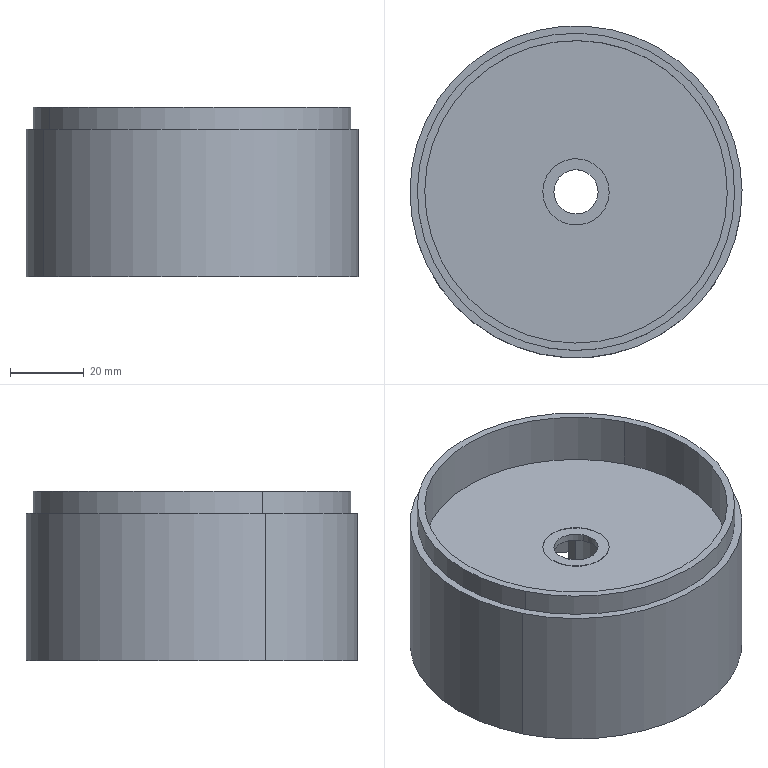Component | SolidWorks | g2-1 | 1 solid | 33 faces | box 90 x 90 x 46 mm | volume 53893 mm3 | cylinder 20 | plane 13 | commonest cylinder face diameters 18 x5 86 x4 82 x4 22 x3 12 x2 90 x2
build123d program:
from build123d import *
from build123d.topology import SkipClean

# Parameters (mm, degrees)
SKETCH1_2_R             = 45
SKETCH1_2_R_2           = 41
BOSS_EXTRUDE1_DEPTH     = 20
BOSS_EXTRUDE2_2_START   = 6
SKETCH2_2_R             = 43
SKETCH2_2_R_2           = 41
BOSS_EXTRUDE2_2_DEPTH   = 6
SKETCH3_W               = 3
SKETCH3_H               = 4.784
SKETCH4_2_W             = 2
SKETCH4_2_H             = 36
BOSS_EXTRUDE3_START     = 16
SKETCH5_R               = 11
SKETCH5_R_2             = 9
BOSS_EXTRUDE3_DEPTH     = 16
BOSS_EXTRUDE4_START     = 2
SKETCH6_R               = 11
SKETCH6_R_2             = 6
BOSS_EXTRUDE4_DEPTH     = 2
CUT_EXTRUDE1_START      = -8
SKETCH1_R               = 43
CUT_EXTRUDE1_DEPTH      = 8
CUT_EXTRUDE2_DEPTH      = 10
CUT_EXTRUDE2_DEPTH_BACK = 10
BOSS_EXTRUDE2_START     = -10
SKETCH4_R               = 9
SKETCH4_R_2             = 6
BOSS_EXTRUDE2_DEPTH     = 1.9


with BuildPart() as part:
    # Sketch1_2 → Boss-Extrude1 (new, symmetric)
    with BuildSketch(Plane.XY):
        Circle(SKETCH1_2_R)
        Circle(SKETCH1_2_R_2, mode=Mode.SUBTRACT)
    extrude(amount=BOSS_EXTRUDE1_DEPTH, both=True)

    # Sketch2_2 → Boss-Extrude2_2 (add)
    with SkipClean():  # the faces are left unmerged after this step: merging them gives an invalid solid
        with BuildSketch(Plane(origin=(0, 0, -20), x_dir=(-1, 0, 0), z_dir=(0, 0, -1)).offset(BOSS_EXTRUDE2_2_START)):
            with Locations(Location((0, 0, 0), (0, 0, 180))):
                Circle(SKETCH2_2_R)
            Circle(SKETCH2_2_R_2, mode=Mode.SUBTRACT)
        extrude(amount=-BOSS_EXTRUDE2_2_DEPTH)

    # Sketch3 → Cut-Revolve2 (revolve, cut)
    with BuildSketch(Plane(origin=(0, 0, 0), x_dir=(0, 0, -1), z_dir=(1, 0, 0)), mode=Mode.PRIVATE) as cut_revolve2_sk:
        with Locations((-18.5, 40.608)):
            Rectangle(SKETCH3_W, SKETCH3_H)
    revolve(cut_revolve2_sk.sketch.rotate(Axis((0, 0, 50.051), (0, 0, -1)), 270), axis=Axis((0, 0, 50.051), (0, 0, -1)), mode=Mode.SUBTRACT)

    # Sketch4_2 → Revolve1 (revolve)
    with BuildSketch(Plane(origin=(0, 0, 0), x_dir=(0, 0, -1), z_dir=(1, 0, 0)), mode=Mode.PRIVATE) as revolve1_sk:
        with Locations((11, 27)):
            Rectangle(SKETCH4_2_W, SKETCH4_2_H)
    revolve(revolve1_sk.sketch.rotate(Axis((0, 0, 44.645), (0, 0, -1)), 270), axis=Axis((0, 0, 44.645), (0, 0, -1)))

    # Sketch5 → Boss-Extrude3 (add)
    with BuildSketch(Plane.XY.offset(-10).offset(BOSS_EXTRUDE3_START)):
        with Locations(Location((0, 0, 0), (0, 0, 180))):
            Circle(SKETCH5_R)
        Circle(SKETCH5_R_2, mode=Mode.SUBTRACT)
    extrude(amount=-BOSS_EXTRUDE3_DEPTH)

    # Sketch6 → Boss-Extrude4 (add)
    with BuildSketch(Plane.XY.offset(6).offset(BOSS_EXTRUDE4_START)):
        with Locations(Location((0, 0, 0), (0, 0, 180))):
            Circle(SKETCH6_R)
        Circle(SKETCH6_R_2, mode=Mode.SUBTRACT)
    extrude(amount=-BOSS_EXTRUDE4_DEPTH)

    # Sketch1 → Cut-Extrude1 (cut)
    with BuildSketch(Plane.XY.offset(20).offset(CUT_EXTRUDE1_START)):
        Circle(SKETCH1_R)
    extrude(amount=CUT_EXTRUDE1_DEPTH, mode=Mode.SUBTRACT)

    # Sketch2 → Cut-Extrude2 (cut, two sides: drawn at the far end of the back side and taken through both)
    with BuildSketch(Plane.XY.offset(-CUT_EXTRUDE2_DEPTH_BACK)):
        Polygon((-18.876, 24.127), (7.766, -29.633), (18.876, -24.127), (-7.766, 29.633), align=None)
    extrude(amount=CUT_EXTRUDE2_DEPTH + CUT_EXTRUDE2_DEPTH_BACK, mode=Mode.SUBTRACT)

    # Sketch4 → Boss-Extrude2 (add)
    with BuildSketch(Plane.XY.offset(BOSS_EXTRUDE2_START)):
        Circle(SKETCH4_R)
        Circle(SKETCH4_R_2, mode=Mode.SUBTRACT)
    extrude(amount=-BOSS_EXTRUDE2_DEPTH)


solid = part.part

# Placed as in the assembly
solid = solid.moved(Location((-15.928, -1.7, 148), (-180, 0, -26.361)))
STEP:
#1=CARTESIAN_POINT('',(-0.4154,0.03795,6.295));
#2=VERTEX_POINT('',#1);
#3=CARTESIAN_POINT('',(-0.8387,-0.1718,6.295));
#4=VERTEX_POINT('',#3);
#5=CARTESIAN_POINT('',(-0.6271,-0.06694,6.295));
#6=DIRECTION('',(0.,0.,-1.));
#7=DIRECTION('',(-0.896,-0.444,0.));
#8=AXIS2_PLACEMENT_3D('',#5,#6,#7);
#9=CIRCLE('',#8,0.2362);
#10=EDGE_CURVE('',#2,#4,#9,.T.);
#11=ORIENTED_EDGE('',*,*,#10,.F.);
#12=CARTESIAN_POINT('',(-0.4154,0.03795,6.22));
#13=VERTEX_POINT('',#12);
#14=CARTESIAN_POINT('',(-0.4154,0.03795,6.295));
#15=DIRECTION('',(0.,0.,-1.));
#16=VECTOR('',#15,39.37);
#17=LINE('',#14,#16);
#18=EDGE_CURVE('',#2,#13,#17,.T.);
#19=ORIENTED_EDGE('',*,*,#18,.T.);
#20=CARTESIAN_POINT('',(-0.8387,-0.1718,6.22));
#21=VERTEX_POINT('',#20);
#22=CARTESIAN_POINT('',(-0.6271,-0.06694,6.22));
#23=DIRECTION('',(0.,0.,-1.));
#24=DIRECTION('',(-0.896,-0.444,0.));
#25=AXIS2_PLACEMENT_3D('',#22,#23,#24);
#26=CIRCLE('',#25,0.2362);
#27=EDGE_CURVE('',#13,#21,#26,.T.);
#28=ORIENTED_EDGE('',*,*,#27,.T.);
#29=CARTESIAN_POINT('',(-0.8387,-0.1718,6.295));
#30=DIRECTION('',(0.,0.,-1.));
#31=VECTOR('',#30,39.37);
#32=LINE('',#29,#31);
#33=EDGE_CURVE('',#4,#21,#32,.T.);
#34=ORIENTED_EDGE('',*,*,#33,.F.);
#35=EDGE_LOOP('',(#11,#19,#28,#34));
#36=FACE_OUTER_BOUND('',#35,.T.);
#37=CARTESIAN_POINT('',(-0.6271,-0.06694,6.295));
#38=DIRECTION('',(0.,0.,-1.));
#39=DIRECTION('',(-0.896,-0.444,0.));
#40=AXIS2_PLACEMENT_3D('',#37,#38,#39);
#41=CYLINDRICAL_SURFACE('',#40,0.2362);
#42=ADVANCED_FACE('',(#36),#41,.F.);
#43=CARTESIAN_POINT('',(0.8898,0.6848,5.354));
#44=VERTEX_POINT('',#43);
#45=CARTESIAN_POINT('',(-2.144,-0.8186,5.354));
#46=VERTEX_POINT('',#45);
#47=CARTESIAN_POINT('',(-0.6271,-0.06694,5.354));
#48=DIRECTION('',(0.,0.,-1.));
#49=DIRECTION('',(-0.896,-0.444,0.));
#50=AXIS2_PLACEMENT_3D('',#47,#48,#49);
#51=CIRCLE('',#50,1.693);
#52=EDGE_CURVE('',#44,#46,#51,.T.);
#53=ORIENTED_EDGE('',*,*,#52,.F.);
#54=CARTESIAN_POINT('',(0.8898,0.6848,5.039));
#55=VERTEX_POINT('',#54);
#56=CARTESIAN_POINT('',(0.8898,0.6848,3.856));
#57=DIRECTION('',(0.,0.,-1.));
#58=VECTOR('',#57,39.37);
#59=LINE('',#56,#58);
#60=EDGE_CURVE('',#44,#55,#59,.T.);
#61=ORIENTED_EDGE('',*,*,#60,.T.);
#62=CARTESIAN_POINT('',(-2.144,-0.8186,5.039));
#63=VERTEX_POINT('',#62);
#64=CARTESIAN_POINT('',(-0.6271,-0.06694,5.039));
#65=DIRECTION('',(0.,0.,-1.));
#66=DIRECTION('',(-0.896,-0.444,0.));
#67=AXIS2_PLACEMENT_3D('',#64,#65,#66);
#68=CIRCLE('',#67,1.693);
#69=EDGE_CURVE('',#55,#63,#68,.T.);
#70=ORIENTED_EDGE('',*,*,#69,.T.);
#71=CARTESIAN_POINT('',(-2.144,-0.8186,3.856));
#72=DIRECTION('',(0.,0.,-1.));
#73=VECTOR('',#72,39.37);
#74=LINE('',#71,#73);
#75=EDGE_CURVE('',#46,#63,#74,.T.);
#76=ORIENTED_EDGE('',*,*,#75,.F.);
#77=EDGE_LOOP('',(#53,#61,#70,#76));
#78=FACE_OUTER_BOUND('',#77,.T.);
#79=CARTESIAN_POINT('',(-0.6271,-0.06694,3.856));
#80=DIRECTION('',(0.,0.,-1.));
#81=DIRECTION('',(-0.896,-0.444,0.));
#82=AXIS2_PLACEMENT_3D('',#79,#80,#81);
#83=CYLINDRICAL_SURFACE('',#82,1.693);
#84=ADVANCED_FACE('',(#78),#83,.F.);
#85=CARTESIAN_POINT('',(0.8898,0.6848,6.85));
#86=VERTEX_POINT('',#85);
#87=CARTESIAN_POINT('',(-2.144,-0.8186,6.85));
#88=VERTEX_POINT('',#87);
#89=CARTESIAN_POINT('',(-0.6271,-0.06694,6.85));
#90=DIRECTION('',(0.,0.,1.));
#91=DIRECTION('',(0.896,0.444,0.));
#92=AXIS2_PLACEMENT_3D('',#89,#90,#91);
#93=CIRCLE('',#92,1.693);
#94=EDGE_CURVE('',#86,#88,#93,.T.);
#95=ORIENTED_EDGE('',*,*,#94,.F.);
#96=CARTESIAN_POINT('',(0.8898,0.6848,6.614));
#97=VERTEX_POINT('',#96);
#98=CARTESIAN_POINT('',(0.8898,0.6848,6.85));
#99=DIRECTION('',(0.,0.,-1.));
#100=VECTOR('',#99,39.37);
#101=LINE('',#98,#100);
#102=EDGE_CURVE('',#86,#97,#101,.T.);
#103=ORIENTED_EDGE('',*,*,#102,.T.);
#104=CARTESIAN_POINT('',(-2.144,-0.8186,6.614));
#105=VERTEX_POINT('',#104);
#106=CARTESIAN_POINT('',(-0.6271,-0.06694,6.614));
#107=DIRECTION('',(0.,0.,1.));
#108=DIRECTION('',(-0.896,-0.444,0.));
#109=AXIS2_PLACEMENT_3D('',#106,#107,#108);
#110=CIRCLE('',#109,1.693);
#111=EDGE_CURVE('',#97,#105,#110,.T.);
#112=ORIENTED_EDGE('',*,*,#111,.T.);
#113=CARTESIAN_POINT('',(-2.144,-0.8186,6.85));
#114=DIRECTION('',(0.,0.,-1.));
#115=VECTOR('',#114,39.37);
#116=LINE('',#113,#115);
#117=EDGE_CURVE('',#88,#105,#116,.T.);
#118=ORIENTED_EDGE('',*,*,#117,.F.);
#119=EDGE_LOOP('',(#95,#103,#112,#118));
#120=FACE_OUTER_BOUND('',#119,.T.);
#121=CARTESIAN_POINT('',(-0.6271,-0.06694,6.85));
#122=DIRECTION('',(0.,0.,-1.));
#123=DIRECTION('',(-0.896,-0.444,0.));
#124=AXIS2_PLACEMENT_3D('',#121,#122,#123);
#125=CYLINDRICAL_SURFACE('',#124,1.693);
#126=ADVANCED_FACE('',(#120),#125,.T.);
#127=CARTESIAN_POINT('',(-2.215,-0.8536,5.039));
#128=VERTEX_POINT('',#127);
#129=CARTESIAN_POINT('',(0.9603,0.7197,5.039));
#130=VERTEX_POINT('',#129);
#131=CARTESIAN_POINT('',(-0.6271,-0.06694,5.039));
#132=DIRECTION('',(0.,0.,-1.));
#133=DIRECTION('',(-0.896,-0.444,0.));
#134=AXIS2_PLACEMENT_3D('',#131,#132,#133);
#135=CIRCLE('',#134,1.772);
#136=EDGE_CURVE('',#128,#130,#135,.T.);
#137=ORIENTED_EDGE('',*,*,#136,.F.);
#138=CARTESIAN_POINT('',(-2.215,-0.8536,6.614));
#139=VERTEX_POINT('',#138);
#140=CARTESIAN_POINT('',(-2.215,-0.8536,5.039));
#141=DIRECTION('',(0.,0.,1.));
#142=VECTOR('',#141,39.37);
#143=LINE('',#140,#142);
#144=EDGE_CURVE('',#128,#139,#143,.T.);
#145=ORIENTED_EDGE('',*,*,#144,.T.);
#146=CARTESIAN_POINT('',(0.9603,0.7197,6.614));
#147=VERTEX_POINT('',#146);
#148=CARTESIAN_POINT('',(-0.6271,-0.06694,6.614));
#149=DIRECTION('',(0.,0.,-1.));
#150=DIRECTION('',(-0.896,-0.444,0.));
#151=AXIS2_PLACEMENT_3D('',#148,#149,#150);
#152=CIRCLE('',#151,1.772);
#153=EDGE_CURVE('',#139,#147,#152,.T.);
#154=ORIENTED_EDGE('',*,*,#153,.T.);
#155=CARTESIAN_POINT('',(0.9603,0.7197,5.039));
#156=DIRECTION('',(0.,0.,1.));
#157=VECTOR('',#156,39.37);
#158=LINE('',#155,#157);
#159=EDGE_CURVE('',#130,#147,#158,.T.);
#160=ORIENTED_EDGE('',*,*,#159,.F.);
#161=EDGE_LOOP('',(#137,#145,#154,#160));
#162=FACE_OUTER_BOUND('',#161,.T.);
#163=CARTESIAN_POINT('',(-0.6271,-0.06694,5.039));
#164=DIRECTION('',(0.,0.,1.));
#165=DIRECTION('',(0.896,0.444,0.));
#166=AXIS2_PLACEMENT_3D('',#163,#164,#165);
#167=CYLINDRICAL_SURFACE('',#166,1.772);
#168=ADVANCED_FACE('',(#162),#167,.T.);
#169=CARTESIAN_POINT('',(0.8192,0.6498,6.299));
#170=VERTEX_POINT('',#169);
#171=CARTESIAN_POINT('',(-2.073,-0.7837,6.299));
#172=VERTEX_POINT('',#171);
#173=CARTESIAN_POINT('',(-0.6271,-0.06694,6.299));
#174=DIRECTION('',(0.,0.,-1.));
#175=DIRECTION('',(-0.896,-0.444,0.));
#176=AXIS2_PLACEMENT_3D('',#173,#174,#175);
#177=CIRCLE('',#176,1.614);
#178=EDGE_CURVE('',#170,#172,#177,.T.);
#179=ORIENTED_EDGE('',*,*,#178,.T.);
#180=CARTESIAN_POINT('',(-2.073,-0.7837,6.85));
#181=VERTEX_POINT('',#180);
#182=CARTESIAN_POINT('',(-2.073,-0.7837,5.039));
#183=DIRECTION('',(0.,0.,1.));
#184=VECTOR('',#183,39.37);
#185=LINE('',#182,#184);
#186=EDGE_CURVE('',#172,#181,#185,.T.);
#187=ORIENTED_EDGE('',*,*,#186,.T.);
#188=CARTESIAN_POINT('',(0.8192,0.6498,6.85));
#189=VERTEX_POINT('',#188);
#190=CARTESIAN_POINT('',(-0.6271,-0.06694,6.85));
#191=DIRECTION('',(0.,0.,1.));
#192=DIRECTION('',(0.896,0.444,0.));
#193=AXIS2_PLACEMENT_3D('',#190,#191,#192);
#194=CIRCLE('',#193,1.614);
#195=EDGE_CURVE('',#181,#189,#194,.T.);
#196=ORIENTED_EDGE('',*,*,#195,.T.);
#197=CARTESIAN_POINT('',(0.8192,0.6498,5.039));
#198=DIRECTION('',(0.,0.,1.));
#199=VECTOR('',#198,39.37);
#200=LINE('',#197,#199);
#201=EDGE_CURVE('',#170,#189,#200,.T.);
#202=ORIENTED_EDGE('',*,*,#201,.F.);
#203=EDGE_LOOP('',(#179,#187,#196,#202));
#204=FACE_OUTER_BOUND('',#203,.T.);
#205=CARTESIAN_POINT('',(-0.6271,-0.06694,5.039));
#206=DIRECTION('',(0.,0.,1.));
#207=DIRECTION('',(0.896,0.444,0.));
#208=AXIS2_PLACEMENT_3D('',#205,#206,#207);
#209=CYLINDRICAL_SURFACE('',#208,1.614);
#210=ADVANCED_FACE('',(#204),#209,.F.);
#211=CARTESIAN_POINT('',(0.8192,0.6498,5.354));
#212=VERTEX_POINT('',#211);
#213=CARTESIAN_POINT('',(-2.073,-0.7837,5.354));
#214=VERTEX_POINT('',#213);
#215=CARTESIAN_POINT('',(-0.6271,-0.06694,5.354));
#216=DIRECTION('',(0.,0.,-1.));
#217=DIRECTION('',(-0.896,-0.444,0.));
#218=AXIS2_PLACEMENT_3D('',#215,#216,#217);
#219=CIRCLE('',#218,1.614);
#220=EDGE_CURVE('',#212,#214,#219,.T.);
#221=ORIENTED_EDGE('',*,*,#220,.T.);
#222=CARTESIAN_POINT('',(-2.073,-0.7837,6.22));
#223=VERTEX_POINT('',#222);
#224=CARTESIAN_POINT('',(-2.073,-0.7837,5.039));
#225=DIRECTION('',(0.,0.,1.));
#226=VECTOR('',#225,39.37);
#227=LINE('',#224,#226);
#228=EDGE_CURVE('',#214,#223,#227,.T.);
#229=ORIENTED_EDGE('',*,*,#228,.T.);
#230=CARTESIAN_POINT('',(0.8192,0.6498,6.22));
#231=VERTEX_POINT('',#230);
#232=CARTESIAN_POINT('',(-0.6271,-0.06694,6.22));
#233=DIRECTION('',(0.,0.,1.));
#234=DIRECTION('',(0.896,0.444,0.));
#235=AXIS2_PLACEMENT_3D('',#232,#233,#234);
#236=CIRCLE('',#235,1.614);
#237=EDGE_CURVE('',#223,#231,#236,.T.);
#238=ORIENTED_EDGE('',*,*,#237,.T.);
#239=CARTESIAN_POINT('',(0.8192,0.6498,5.039));
#240=DIRECTION('',(0.,0.,1.));
#241=VECTOR('',#240,39.37);
#242=LINE('',#239,#241);
#243=EDGE_CURVE('',#212,#231,#242,.T.);
#244=ORIENTED_EDGE('',*,*,#243,.F.);
#245=EDGE_LOOP('',(#221,#229,#238,#244));
#246=FACE_OUTER_BOUND('',#245,.T.);
#247=CARTESIAN_POINT('',(-0.6271,-0.06694,5.039));
#248=DIRECTION('',(0.,0.,1.));
#249=DIRECTION('',(0.896,0.444,0.));
#250=AXIS2_PLACEMENT_3D('',#247,#248,#249);
#251=CYLINDRICAL_SURFACE('',#250,1.614);
#252=ADVANCED_FACE('',(#246),#251,.F.);
#253=CARTESIAN_POINT('',(-0.2391,0.1254,5.512));
#254=VERTEX_POINT('',#253);
#255=CARTESIAN_POINT('',(-0.383,-0.4247,5.512));
#256=VERTEX_POINT('',#255);
#257=CARTESIAN_POINT('',(-0.6271,-0.06694,5.512));
#258=DIRECTION('',(0.,0.,-1.));
#259=DIRECTION('',(-0.896,-0.444,0.));
#260=AXIS2_PLACEMENT_3D('',#257,#258,#259);
#261=CIRCLE('',#260,0.4331);
#262=EDGE_CURVE('',#254,#256,#261,.T.);
#263=ORIENTED_EDGE('',*,*,#262,.F.);
#264=CARTESIAN_POINT('',(-0.2391,0.1254,6.22));
#265=VERTEX_POINT('',#264);
#266=CARTESIAN_POINT('',(-0.2391,0.1254,5.591));
#267=DIRECTION('',(0.,0.,1.));
#268=VECTOR('',#267,39.37);
#269=LINE('',#266,#268);
#270=EDGE_CURVE('',#254,#265,#269,.T.);
#271=ORIENTED_EDGE('',*,*,#270,.T.);
#272=CARTESIAN_POINT('',(-0.383,-0.4247,6.22));
#273=VERTEX_POINT('',#272);
#274=CARTESIAN_POINT('',(-0.6271,-0.06694,6.22));
#275=DIRECTION('',(0.,0.,-1.));
#276=DIRECTION('',(0.896,0.444,0.));
#277=AXIS2_PLACEMENT_3D('',#274,#275,#276);
#278=CIRCLE('',#277,0.4331);
#279=EDGE_CURVE('',#265,#273,#278,.T.);
#280=ORIENTED_EDGE('',*,*,#279,.T.);
#281=CARTESIAN_POINT('',(-0.383,-0.4247,5.591));
#282=DIRECTION('',(0.,0.,1.));
#283=VECTOR('',#282,39.37);
#284=LINE('',#281,#283);
#285=EDGE_CURVE('',#256,#273,#284,.T.);
#286=ORIENTED_EDGE('',*,*,#285,.F.);
#287=EDGE_LOOP('',(#263,#271,#280,#286));
#288=FACE_OUTER_BOUND('',#287,.T.);
#289=CARTESIAN_POINT('',(-0.6271,-0.06694,5.591));
#290=DIRECTION('',(0.,0.,1.));
#291=DIRECTION('',(0.896,0.444,0.));
#292=AXIS2_PLACEMENT_3D('',#289,#290,#291);
#293=CYLINDRICAL_SURFACE('',#292,0.4331);
#294=ADVANCED_FACE('',(#288),#293,.T.);
#295=CARTESIAN_POINT('',(-0.3096,0.0904,6.299));
#296=VERTEX_POINT('',#295);
#297=CARTESIAN_POINT('',(-0.9446,-0.2243,6.299));
#298=VERTEX_POINT('',#297);
#299=CARTESIAN_POINT('',(-0.6271,-0.06694,6.299));
#300=DIRECTION('',(0.,0.,-1.));
#301=DIRECTION('',(-0.896,-0.444,0.));
#302=AXIS2_PLACEMENT_3D('',#299,#300,#301);
#303=CIRCLE('',#302,0.3543);
#304=EDGE_CURVE('',#296,#298,#303,.T.);
#305=ORIENTED_EDGE('',*,*,#304,.F.);
#306=CARTESIAN_POINT('',(-0.3096,0.0904,6.295));
#307=VERTEX_POINT('',#306);
#308=CARTESIAN_POINT('',(-0.3096,0.0904,4.069));
#309=DIRECTION('',(0.,0.,-1.));
#310=VECTOR('',#309,39.37);
#311=LINE('',#308,#310);
#312=EDGE_CURVE('',#296,#307,#311,.T.);
#313=ORIENTED_EDGE('',*,*,#312,.T.);
#314=CARTESIAN_POINT('',(-0.9446,-0.2243,6.295));
#315=VERTEX_POINT('',#314);
#316=CARTESIAN_POINT('',(-0.6271,-0.06694,6.295));
#317=DIRECTION('',(0.,0.,1.));
#318=DIRECTION('',(-0.896,-0.444,0.));
#319=AXIS2_PLACEMENT_3D('',#316,#317,#318);
#320=CIRCLE('',#319,0.3543);
#321=EDGE_CURVE('',#315,#307,#320,.T.);
#322=ORIENTED_EDGE('',*,*,#321,.F.);
#323=CARTESIAN_POINT('',(-0.9446,-0.2243,4.069));
#324=DIRECTION('',(0.,0.,-1.));
#325=VECTOR('',#324,39.37);
#326=LINE('',#323,#325);
#327=EDGE_CURVE('',#298,#315,#326,.T.);
#328=ORIENTED_EDGE('',*,*,#327,.F.);
#329=EDGE_LOOP('',(#305,#313,#322,#328));
#330=FACE_OUTER_BOUND('',#329,.T.);
#331=CARTESIAN_POINT('',(-0.6271,-0.06694,4.069));
#332=DIRECTION('',(0.,0.,-1.));
#333=DIRECTION('',(-0.896,-0.444,0.));
#334=AXIS2_PLACEMENT_3D('',#331,#332,#333);
#335=CYLINDRICAL_SURFACE('',#334,0.3543);
#336=ADVANCED_FACE('',(#330),#335,.F.);
#337=CARTESIAN_POINT('',(-0.9446,-0.2243,6.22));
#338=VERTEX_POINT('',#337);
#339=CARTESIAN_POINT('',(-0.8712,0.1899,6.22));
#340=VERTEX_POINT('',#339);
#341=CARTESIAN_POINT('',(-0.6271,-0.06694,6.22));
#342=DIRECTION('',(0.,0.,-1.));
#343=DIRECTION('',(-0.896,-0.444,0.));
#344=AXIS2_PLACEMENT_3D('',#341,#342,#343);
#345=CIRCLE('',#344,0.3543);
#346=EDGE_CURVE('',#338,#340,#345,.T.);
#347=ORIENTED_EDGE('',*,*,#346,.F.);
#348=CARTESIAN_POINT('',(-0.9446,-0.2243,5.591));
#349=VERTEX_POINT('',#348);
#350=CARTESIAN_POINT('',(-0.9446,-0.2243,4.069));
#351=DIRECTION('',(0.,0.,-1.));
#352=VECTOR('',#351,39.37);
#353=LINE('',#350,#352);
#354=EDGE_CURVE('',#338,#349,#353,.T.);
#355=ORIENTED_EDGE('',*,*,#354,.T.);
#356=CARTESIAN_POINT('',(-0.8712,0.1899,5.591));
#357=VERTEX_POINT('',#356);
#358=CARTESIAN_POINT('',(-0.6271,-0.06694,5.591));
#359=DIRECTION('',(0.,0.,1.));
#360=DIRECTION('',(-0.896,-0.444,0.));
#361=AXIS2_PLACEMENT_3D('',#358,#359,#360);
#362=CIRCLE('',#361,0.3543);
#363=EDGE_CURVE('',#357,#349,#362,.T.);
#364=ORIENTED_EDGE('',*,*,#363,.F.);
#365=CARTESIAN_POINT('',(-0.8712,0.1899,4.069));
#366=DIRECTION('',(0.,0.,-1.));
#367=VECTOR('',#366,39.37);
#368=LINE('',#365,#367);
#369=EDGE_CURVE('',#340,#357,#368,.T.);
#370=ORIENTED_EDGE('',*,*,#369,.F.);
#371=EDGE_LOOP('',(#347,#355,#364,#370));
#372=FACE_OUTER_BOUND('',#371,.T.);
#373=CARTESIAN_POINT('',(-0.6271,-0.06694,4.069));
#374=DIRECTION('',(0.,0.,-1.));
#375=DIRECTION('',(-0.896,-0.444,0.));
#376=AXIS2_PLACEMENT_3D('',#373,#374,#375);
#377=CYLINDRICAL_SURFACE('',#376,0.3543);
#378=ADVANCED_FACE('',(#372),#377,.F.);
#379=CARTESIAN_POINT('',(-0.383,0.1899,6.22));
#380=VERTEX_POINT('',#379);
#381=CARTESIAN_POINT('',(-0.383,-0.3238,6.22));
#382=VERTEX_POINT('',#381);
#383=CARTESIAN_POINT('',(-0.6271,-0.06694,6.22));
#384=DIRECTION('',(0.,0.,-1.));
#385=DIRECTION('',(-0.896,-0.444,0.));
#386=AXIS2_PLACEMENT_3D('',#383,#384,#385);
#387=CIRCLE('',#386,0.3543);
#388=EDGE_CURVE('',#380,#382,#387,.T.);
#389=ORIENTED_EDGE('',*,*,#388,.F.);
#390=CARTESIAN_POINT('',(-0.383,0.1899,5.591));
#391=VERTEX_POINT('',#390);
#392=CARTESIAN_POINT('',(-0.383,0.1899,4.069));
#393=DIRECTION('',(0.,0.,1.));
#394=VECTOR('',#393,39.37);
#395=LINE('',#392,#394);
#396=EDGE_CURVE('',#391,#380,#395,.T.);
#397=ORIENTED_EDGE('',*,*,#396,.F.);
#398=CARTESIAN_POINT('',(-0.383,-0.3238,5.591));
#399=VERTEX_POINT('',#398);
#400=CARTESIAN_POINT('',(-0.6271,-0.06694,5.591));
#401=DIRECTION('',(0.,0.,1.));
#402=DIRECTION('',(-0.896,-0.444,0.));
#403=AXIS2_PLACEMENT_3D('',#400,#401,#402);
#404=CIRCLE('',#403,0.3543);
#405=EDGE_CURVE('',#399,#391,#404,.T.);
#406=ORIENTED_EDGE('',*,*,#405,.F.);
#407=CARTESIAN_POINT('',(-0.383,-0.3238,4.069));
#408=DIRECTION('',(0.,0.,-1.));
#409=VECTOR('',#408,39.37);
#410=LINE('',#407,#409);
#411=EDGE_CURVE('',#382,#399,#410,.T.);
#412=ORIENTED_EDGE('',*,*,#411,.F.);
#413=EDGE_LOOP('',(#389,#397,#406,#412));
#414=FACE_OUTER_BOUND('',#413,.T.);
#415=CARTESIAN_POINT('',(-0.6271,-0.06694,4.069));
#416=DIRECTION('',(0.,0.,-1.));
#417=DIRECTION('',(-0.896,-0.444,0.));
#418=AXIS2_PLACEMENT_3D('',#415,#416,#417);
#419=CYLINDRICAL_SURFACE('',#418,0.3543);
#420=ADVANCED_FACE('',(#414),#419,.F.);
#421=ORIENTED_EDGE('',*,*,#354,.F.);
#422=CARTESIAN_POINT('',(-0.8712,-0.3238,6.22));
#423=VERTEX_POINT('',#422);
#424=CARTESIAN_POINT('',(-0.6271,-0.06694,6.22));
#425=DIRECTION('',(0.,0.,-1.));
#426=DIRECTION('',(-0.896,-0.444,0.));
#427=AXIS2_PLACEMENT_3D('',#424,#425,#426);
#428=CIRCLE('',#427,0.3543);
#429=EDGE_CURVE('',#423,#338,#428,.T.);
#430=ORIENTED_EDGE('',*,*,#429,.F.);
#431=CARTESIAN_POINT('',(-0.8712,-0.3238,5.591));
#432=VERTEX_POINT('',#431);
#433=CARTESIAN_POINT('',(-0.8712,-0.3238,4.069));
#434=DIRECTION('',(0.,0.,1.));
#435=VECTOR('',#434,39.37);
#436=LINE('',#433,#435);
#437=EDGE_CURVE('',#432,#423,#436,.T.);
#438=ORIENTED_EDGE('',*,*,#437,.F.);
#439=CARTESIAN_POINT('',(-0.6271,-0.06694,5.591));
#440=DIRECTION('',(0.,0.,1.));
#441=DIRECTION('',(-0.896,-0.444,0.));
#442=AXIS2_PLACEMENT_3D('',#439,#440,#441);
#443=CIRCLE('',#442,0.3543);
#444=EDGE_CURVE('',#349,#432,#443,.T.);
#445=ORIENTED_EDGE('',*,*,#444,.F.);
#446=EDGE_LOOP('',(#421,#430,#438,#445));
#447=FACE_OUTER_BOUND('',#446,.T.);
#448=CARTESIAN_POINT('',(-0.6271,-0.06694,4.069));
#449=DIRECTION('',(0.,0.,-1.));
#450=DIRECTION('',(-0.896,-0.444,0.));
#451=AXIS2_PLACEMENT_3D('',#448,#449,#450);
#452=CYLINDRICAL_SURFACE('',#451,0.3543);
#453=ADVANCED_FACE('',(#447),#452,.F.);
#454=ORIENTED_EDGE('',*,*,#312,.F.);
#455=CARTESIAN_POINT('',(-0.6271,-0.06694,6.299));
#456=DIRECTION('',(0.,0.,-1.));
#457=DIRECTION('',(-0.896,-0.444,0.));
#458=AXIS2_PLACEMENT_3D('',#455,#456,#457);
#459=CIRCLE('',#458,0.3543);
#460=EDGE_CURVE('',#298,#296,#459,.T.);
#461=ORIENTED_EDGE('',*,*,#460,.F.);
#462=ORIENTED_EDGE('',*,*,#327,.T.);
#463=CARTESIAN_POINT('',(-0.6271,-0.06694,6.295));
#464=DIRECTION('',(0.,0.,1.));
#465=DIRECTION('',(-0.896,-0.444,0.));
#466=AXIS2_PLACEMENT_3D('',#463,#464,#465);
#467=CIRCLE('',#466,0.3543);
#468=EDGE_CURVE('',#307,#315,#467,.T.);
#469=ORIENTED_EDGE('',*,*,#468,.F.);
#470=EDGE_LOOP('',(#454,#461,#462,#469));
#471=FACE_OUTER_BOUND('',#470,.T.);
#472=CARTESIAN_POINT('',(-0.6271,-0.06694,4.069));
#473=DIRECTION('',(0.,0.,-1.));
#474=DIRECTION('',(-0.896,-0.444,0.));
#475=AXIS2_PLACEMENT_3D('',#472,#473,#474);
#476=CYLINDRICAL_SURFACE('',#475,0.3543);
#477=ADVANCED_FACE('',(#471),#476,.F.);
#478=ORIENTED_EDGE('',*,*,#270,.F.);
#479=CARTESIAN_POINT('',(-0.383,0.2908,5.512));
#480=VERTEX_POINT('',#479);
#481=CARTESIAN_POINT('',(-0.6271,-0.06694,5.512));
#482=DIRECTION('',(0.,0.,-1.));
#483=DIRECTION('',(-0.896,-0.444,0.));
#484=AXIS2_PLACEMENT_3D('',#481,#482,#483);
#485=CIRCLE('',#484,0.4331);
#486=EDGE_CURVE('',#480,#254,#485,.T.);
#487=ORIENTED_EDGE('',*,*,#486,.F.);
#488=CARTESIAN_POINT('',(-0.383,0.2908,6.22));
#489=VERTEX_POINT('',#488);
#490=CARTESIAN_POINT('',(-0.383,0.2908,5.591));
#491=DIRECTION('',(0.,0.,-1.));
#492=VECTOR('',#491,39.37);
#493=LINE('',#490,#492);
#494=EDGE_CURVE('',#489,#480,#493,.T.);
#495=ORIENTED_EDGE('',*,*,#494,.F.);
#496=CARTESIAN_POINT('',(-0.6271,-0.06694,6.22));
#497=DIRECTION('',(0.,0.,-1.));
#498=DIRECTION('',(0.896,0.444,0.));
#499=AXIS2_PLACEMENT_3D('',#496,#497,#498);
#500=CIRCLE('',#499,0.4331);
#501=EDGE_CURVE('',#489,#265,#500,.T.);
#502=ORIENTED_EDGE('',*,*,#501,.T.);
#503=EDGE_LOOP('',(#478,#487,#495,#502));
#504=FACE_OUTER_BOUND('',#503,.T.);
#505=CARTESIAN_POINT('',(-0.6271,-0.06694,5.591));
#506=DIRECTION('',(0.,0.,1.));
#507=DIRECTION('',(0.896,0.444,0.));
#508=AXIS2_PLACEMENT_3D('',#505,#506,#507);
#509=CYLINDRICAL_SURFACE('',#508,0.4331);
#510=ADVANCED_FACE('',(#504),#509,.T.);
#511=CARTESIAN_POINT('',(-0.8712,0.2908,5.512));
#512=VERTEX_POINT('',#511);
#513=CARTESIAN_POINT('',(-0.8712,0.2908,6.22));
#514=VERTEX_POINT('',#513);
#515=CARTESIAN_POINT('',(-0.8712,0.2908,5.591));
#516=DIRECTION('',(0.,0.,1.));
#517=VECTOR('',#516,39.37);
#518=LINE('',#515,#517);
#519=EDGE_CURVE('',#512,#514,#518,.T.);
#520=ORIENTED_EDGE('',*,*,#519,.F.);
#521=CARTESIAN_POINT('',(-0.8712,-0.4247,5.512));
#522=VERTEX_POINT('',#521);
#523=CARTESIAN_POINT('',(-0.6271,-0.06694,5.512));
#524=DIRECTION('',(0.,0.,-1.));
#525=DIRECTION('',(-0.896,-0.444,0.));
#526=AXIS2_PLACEMENT_3D('',#523,#524,#525);
#527=CIRCLE('',#526,0.4331);
#528=EDGE_CURVE('',#522,#512,#527,.T.);
#529=ORIENTED_EDGE('',*,*,#528,.F.);
#530=CARTESIAN_POINT('',(-0.8712,-0.4247,6.22));
#531=VERTEX_POINT('',#530);
#532=CARTESIAN_POINT('',(-0.8712,-0.4247,5.591));
#533=DIRECTION('',(0.,0.,-1.));
#534=VECTOR('',#533,39.37);
#535=LINE('',#532,#534);
#536=EDGE_CURVE('',#531,#522,#535,.T.);
#537=ORIENTED_EDGE('',*,*,#536,.F.);
#538=CARTESIAN_POINT('',(-0.6271,-0.06694,6.22));
#539=DIRECTION('',(0.,0.,-1.));
#540=DIRECTION('',(0.896,0.444,0.));
#541=AXIS2_PLACEMENT_3D('',#538,#539,#540);
#542=CIRCLE('',#541,0.4331);
#543=EDGE_CURVE('',#531,#514,#542,.T.);
#544=ORIENTED_EDGE('',*,*,#543,.T.);
#545=EDGE_LOOP('',(#520,#529,#537,#544));
#546=FACE_OUTER_BOUND('',#545,.T.);
#547=CARTESIAN_POINT('',(-0.6271,-0.06694,5.591));
#548=DIRECTION('',(0.,0.,1.));
#549=DIRECTION('',(0.896,0.444,0.));
#550=AXIS2_PLACEMENT_3D('',#547,#548,#549);
#551=CYLINDRICAL_SURFACE('',#550,0.4331);
#552=ADVANCED_FACE('',(#546),#551,.T.);
#553=CARTESIAN_POINT('',(-0.383,-0.06694,5.591));
#554=DIRECTION('',(0.,1.,0.));
#555=VECTOR('',#554,39.37);
#556=LINE('',#553,#555);
#557=EDGE_CURVE('',#399,#391,#556,.T.);
#558=ORIENTED_EDGE('',*,*,#557,.F.);
#559=ORIENTED_EDGE('',*,*,#405,.T.);
#560=EDGE_LOOP('',(#558,#559));
#561=FACE_OUTER_BOUND('',#560,.T.);
#562=CARTESIAN_POINT('',(-0.6271,-0.06694,5.591));
#563=DIRECTION('',(0.,0.,-1.));
#564=DIRECTION('',(-0.896,-0.444,0.));
#565=AXIS2_PLACEMENT_3D('',#562,#563,#564);
#566=PLANE('',#565);
#567=ADVANCED_FACE('',(#561),#566,.F.);
#568=CARTESIAN_POINT('',(-0.8712,-0.06694,5.591));
#569=DIRECTION('',(-0.,-1.,0.));
#570=VECTOR('',#569,39.37);
#571=LINE('',#568,#570);
#572=EDGE_CURVE('',#357,#432,#571,.T.);
#573=ORIENTED_EDGE('',*,*,#572,.F.);
#574=ORIENTED_EDGE('',*,*,#363,.T.);
#575=ORIENTED_EDGE('',*,*,#444,.T.);
#576=EDGE_LOOP('',(#573,#574,#575));
#577=FACE_OUTER_BOUND('',#576,.T.);
#578=CARTESIAN_POINT('',(-0.6271,-0.06694,5.591));
#579=DIRECTION('',(0.,0.,-1.));
#580=DIRECTION('',(-0.896,-0.444,0.));
#581=AXIS2_PLACEMENT_3D('',#578,#579,#580);
#582=PLANE('',#581);
#583=ADVANCED_FACE('',(#577),#582,.F.);
#584=ORIENTED_EDGE('',*,*,#486,.T.);
#585=ORIENTED_EDGE('',*,*,#262,.T.);
#586=CARTESIAN_POINT('',(-0.383,-0.06694,5.512));
#587=DIRECTION('',(0.,1.,0.));
#588=VECTOR('',#587,39.37);
#589=LINE('',#586,#588);
#590=EDGE_CURVE('',#256,#480,#589,.T.);
#591=ORIENTED_EDGE('',*,*,#590,.T.);
#592=EDGE_LOOP('',(#584,#585,#591));
#593=FACE_OUTER_BOUND('',#592,.T.);
#594=CARTESIAN_POINT('',(-0.6271,-0.06694,5.512));
#595=DIRECTION('',(0.,0.,-1.));
#596=DIRECTION('',(-0.896,-0.444,0.));
#597=AXIS2_PLACEMENT_3D('',#594,#595,#596);
#598=PLANE('',#597);
#599=ADVANCED_FACE('',(#593),#598,.T.);
#600=ORIENTED_EDGE('',*,*,#528,.T.);
#601=CARTESIAN_POINT('',(-0.8712,-0.06694,5.512));
#602=DIRECTION('',(-0.,-1.,0.));
#603=VECTOR('',#602,39.37);
#604=LINE('',#601,#603);
#605=EDGE_CURVE('',#512,#522,#604,.T.);
#606=ORIENTED_EDGE('',*,*,#605,.T.);
#607=EDGE_LOOP('',(#600,#606));
#608=FACE_OUTER_BOUND('',#607,.T.);
#609=CARTESIAN_POINT('',(-0.6271,-0.06694,5.512));
#610=DIRECTION('',(0.,0.,-1.));
#611=DIRECTION('',(-0.896,-0.444,0.));
#612=AXIS2_PLACEMENT_3D('',#609,#610,#611);
#613=PLANE('',#612);
#614=ADVANCED_FACE('',(#608),#613,.T.);
#615=ORIENTED_EDGE('',*,*,#228,.F.);
#616=CARTESIAN_POINT('',(-0.6271,-0.06694,5.354));
#617=DIRECTION('',(0.,0.,-1.));
#618=DIRECTION('',(-0.896,-0.444,0.));
#619=AXIS2_PLACEMENT_3D('',#616,#617,#618);
#620=CIRCLE('',#619,1.614);
#621=EDGE_CURVE('',#214,#212,#620,.T.);
#622=ORIENTED_EDGE('',*,*,#621,.T.);
#623=ORIENTED_EDGE('',*,*,#243,.T.);
#624=CARTESIAN_POINT('',(-0.6271,-0.06694,6.22));
#625=DIRECTION('',(0.,0.,1.));
#626=DIRECTION('',(0.896,0.444,0.));
#627=AXIS2_PLACEMENT_3D('',#624,#625,#626);
#628=CIRCLE('',#627,1.614);
#629=EDGE_CURVE('',#231,#223,#628,.T.);
#630=ORIENTED_EDGE('',*,*,#629,.T.);
#631=EDGE_LOOP('',(#615,#622,#623,#630));
#632=FACE_OUTER_BOUND('',#631,.T.);
#633=CARTESIAN_POINT('',(-0.6271,-0.06694,5.039));
#634=DIRECTION('',(0.,0.,1.));
#635=DIRECTION('',(0.896,0.444,0.));
#636=AXIS2_PLACEMENT_3D('',#633,#634,#635);
#637=CYLINDRICAL_SURFACE('',#636,1.614);
#638=ADVANCED_FACE('',(#632),#637,.F.);
#639=ORIENTED_EDGE('',*,*,#429,.T.);
#640=ORIENTED_EDGE('',*,*,#346,.T.);
#641=CARTESIAN_POINT('',(-0.8712,-1.248,6.22));
#642=DIRECTION('',(0.,1.,0.));
#643=VECTOR('',#642,39.37);
#644=LINE('',#641,#643);
#645=EDGE_CURVE('',#340,#514,#644,.T.);
#646=ORIENTED_EDGE('',*,*,#645,.T.);
#647=ORIENTED_EDGE('',*,*,#543,.F.);
#648=CARTESIAN_POINT('',(-0.8712,-1.248,6.22));
#649=DIRECTION('',(0.,1.,0.));
#650=VECTOR('',#649,39.37);
#651=LINE('',#648,#650);
#652=EDGE_CURVE('',#531,#423,#651,.T.);
#653=ORIENTED_EDGE('',*,*,#652,.T.);
#654=EDGE_LOOP('',(#639,#640,#646,#647,#653));
#655=FACE_BOUND('',#654,.T.);
#656=CARTESIAN_POINT('',(-0.383,1.114,6.22));
#657=DIRECTION('',(0.,-1.,0.));
#658=VECTOR('',#657,39.37);
#659=LINE('',#656,#658);
#660=EDGE_CURVE('',#489,#380,#659,.T.);
#661=ORIENTED_EDGE('',*,*,#660,.T.);
#662=ORIENTED_EDGE('',*,*,#388,.T.);
#663=CARTESIAN_POINT('',(-0.383,1.114,6.22));
#664=DIRECTION('',(0.,-1.,0.));
#665=VECTOR('',#664,39.37);
#666=LINE('',#663,#665);
#667=EDGE_CURVE('',#382,#273,#666,.T.);
#668=ORIENTED_EDGE('',*,*,#667,.T.);
#669=ORIENTED_EDGE('',*,*,#279,.F.);
#670=ORIENTED_EDGE('',*,*,#501,.F.);
#671=EDGE_LOOP('',(#661,#662,#668,#669,#670));
#672=FACE_BOUND('',#671,.T.);
#673=ORIENTED_EDGE('',*,*,#629,.F.);
#674=ORIENTED_EDGE('',*,*,#237,.F.);
#675=EDGE_LOOP('',(#673,#674));
#676=FACE_OUTER_BOUND('',#675,.T.);
#677=CARTESIAN_POINT('',(-0.6271,-0.06694,6.22));
#678=DIRECTION('',(0.,0.,-1.));
#679=DIRECTION('',(-0.896,-0.444,0.));
#680=AXIS2_PLACEMENT_3D('',#677,#678,#679);
#681=CIRCLE('',#680,0.2362);
#682=EDGE_CURVE('',#21,#13,#681,.T.);
#683=ORIENTED_EDGE('',*,*,#682,.F.);
#684=ORIENTED_EDGE('',*,*,#27,.F.);
#685=EDGE_LOOP('',(#683,#684));
#686=FACE_BOUND('',#685,.T.);
#687=CARTESIAN_POINT('',(-1.414,1.52,6.22));
#688=DIRECTION('',(0.,0.,1.));
#689=DIRECTION('',(0.896,0.444,0.));
#690=AXIS2_PLACEMENT_3D('',#687,#688,#689);
#691=PLANE('',#690);
#692=ADVANCED_FACE('',(#655,#672,#676,#686),#691,.F.);
#693=ORIENTED_EDGE('',*,*,#186,.F.);
#694=CARTESIAN_POINT('',(-0.6271,-0.06694,6.299));
#695=DIRECTION('',(0.,0.,-1.));
#696=DIRECTION('',(-0.896,-0.444,0.));
#697=AXIS2_PLACEMENT_3D('',#694,#695,#696);
#698=CIRCLE('',#697,1.614);
#699=EDGE_CURVE('',#172,#170,#698,.T.);
#700=ORIENTED_EDGE('',*,*,#699,.T.);
#701=ORIENTED_EDGE('',*,*,#201,.T.);
#702=CARTESIAN_POINT('',(-0.6271,-0.06694,6.85));
#703=DIRECTION('',(0.,0.,1.));
#704=DIRECTION('',(0.896,0.444,0.));
#705=AXIS2_PLACEMENT_3D('',#702,#703,#704);
#706=CIRCLE('',#705,1.614);
#707=EDGE_CURVE('',#189,#181,#706,.T.);
#708=ORIENTED_EDGE('',*,*,#707,.T.);
#709=EDGE_LOOP('',(#693,#700,#701,#708));
#710=FACE_OUTER_BOUND('',#709,.T.);
#711=CARTESIAN_POINT('',(-0.6271,-0.06694,5.039));
#712=DIRECTION('',(0.,0.,1.));
#713=DIRECTION('',(0.896,0.444,0.));
#714=AXIS2_PLACEMENT_3D('',#711,#712,#713);
#715=CYLINDRICAL_SURFACE('',#714,1.614);
#716=ADVANCED_FACE('',(#710),#715,.F.);
#717=CARTESIAN_POINT('',(-0.6271,-0.06694,5.039));
#718=DIRECTION('',(0.,0.,-1.));
#719=DIRECTION('',(-0.896,-0.444,0.));
#720=AXIS2_PLACEMENT_3D('',#717,#718,#719);
#721=CIRCLE('',#720,1.772);
#722=EDGE_CURVE('',#130,#128,#721,.T.);
#723=ORIENTED_EDGE('',*,*,#722,.T.);
#724=ORIENTED_EDGE('',*,*,#136,.T.);
#725=EDGE_LOOP('',(#723,#724));
#726=FACE_OUTER_BOUND('',#725,.T.);
#727=CARTESIAN_POINT('',(-0.6271,-0.06694,5.039));
#728=DIRECTION('',(0.,0.,-1.));
#729=DIRECTION('',(-0.896,-0.444,0.));
#730=AXIS2_PLACEMENT_3D('',#727,#728,#729);
#731=CIRCLE('',#730,1.693);
#732=EDGE_CURVE('',#63,#55,#731,.T.);
#733=ORIENTED_EDGE('',*,*,#732,.F.);
#734=ORIENTED_EDGE('',*,*,#69,.F.);
#735=EDGE_LOOP('',(#733,#734));
#736=FACE_BOUND('',#735,.T.);
#737=CARTESIAN_POINT('',(-0.6271,-0.06694,5.039));
#738=DIRECTION('',(0.,0.,-1.));
#739=DIRECTION('',(-0.896,-0.444,0.));
#740=AXIS2_PLACEMENT_3D('',#737,#738,#739);
#741=PLANE('',#740);
#742=ADVANCED_FACE('',(#726,#736),#741,.T.);
#743=CARTESIAN_POINT('',(-0.6271,-0.06694,6.614));
#744=DIRECTION('',(0.,0.,-1.));
#745=DIRECTION('',(-0.896,-0.444,0.));
#746=AXIS2_PLACEMENT_3D('',#743,#744,#745);
#747=CIRCLE('',#746,1.772);
#748=EDGE_CURVE('',#147,#139,#747,.T.);
#749=ORIENTED_EDGE('',*,*,#748,.F.);
#750=ORIENTED_EDGE('',*,*,#153,.F.);
#751=EDGE_LOOP('',(#749,#750));
#752=FACE_OUTER_BOUND('',#751,.T.);
#753=CARTESIAN_POINT('',(-0.6271,-0.06694,6.614));
#754=DIRECTION('',(0.,0.,1.));
#755=DIRECTION('',(-0.896,-0.444,0.));
#756=AXIS2_PLACEMENT_3D('',#753,#754,#755);
#757=CIRCLE('',#756,1.693);
#758=EDGE_CURVE('',#105,#97,#757,.T.);
#759=ORIENTED_EDGE('',*,*,#758,.F.);
#760=ORIENTED_EDGE('',*,*,#111,.F.);
#761=EDGE_LOOP('',(#759,#760));
#762=FACE_BOUND('',#761,.T.);
#763=CARTESIAN_POINT('',(-0.6271,-0.06694,6.614));
#764=DIRECTION('',(0.,0.,-1.));
#765=DIRECTION('',(-0.896,-0.444,0.));
#766=AXIS2_PLACEMENT_3D('',#763,#764,#765);
#767=PLANE('',#766);
#768=ADVANCED_FACE('',(#752,#762),#767,.F.);
#769=ORIENTED_EDGE('',*,*,#144,.F.);
#770=ORIENTED_EDGE('',*,*,#722,.F.);
#771=ORIENTED_EDGE('',*,*,#159,.T.);
#772=ORIENTED_EDGE('',*,*,#748,.T.);
#773=EDGE_LOOP('',(#769,#770,#771,#772));
#774=FACE_OUTER_BOUND('',#773,.T.);
#775=CARTESIAN_POINT('',(-0.6271,-0.06694,5.039));
#776=DIRECTION('',(0.,0.,1.));
#777=DIRECTION('',(0.896,0.444,0.));
#778=AXIS2_PLACEMENT_3D('',#775,#776,#777);
#779=CYLINDRICAL_SURFACE('',#778,1.772);
#780=ADVANCED_FACE('',(#774),#779,.T.);
#781=CARTESIAN_POINT('',(-0.6271,-0.06694,6.85));
#782=DIRECTION('',(0.,0.,1.));
#783=DIRECTION('',(0.896,0.444,0.));
#784=AXIS2_PLACEMENT_3D('',#781,#782,#783);
#785=CIRCLE('',#784,1.693);
#786=EDGE_CURVE('',#88,#86,#785,.T.);
#787=ORIENTED_EDGE('',*,*,#786,.T.);
#788=ORIENTED_EDGE('',*,*,#94,.T.);
#789=EDGE_LOOP('',(#787,#788));
#790=FACE_OUTER_BOUND('',#789,.T.);
#791=ORIENTED_EDGE('',*,*,#707,.F.);
#792=ORIENTED_EDGE('',*,*,#195,.F.);
#793=EDGE_LOOP('',(#791,#792));
#794=FACE_BOUND('',#793,.T.);
#795=CARTESIAN_POINT('',(-0.6271,-0.06694,6.85));
#796=DIRECTION('',(0.,0.,1.));
#797=DIRECTION('',(0.896,0.444,0.));
#798=AXIS2_PLACEMENT_3D('',#795,#796,#797);
#799=PLANE('',#798);
#800=ADVANCED_FACE('',(#790,#794),#799,.T.);
#801=ORIENTED_EDGE('',*,*,#102,.F.);
#802=ORIENTED_EDGE('',*,*,#786,.F.);
#803=ORIENTED_EDGE('',*,*,#117,.T.);
#804=ORIENTED_EDGE('',*,*,#758,.T.);
#805=EDGE_LOOP('',(#801,#802,#803,#804));
#806=FACE_OUTER_BOUND('',#805,.T.);
#807=CARTESIAN_POINT('',(-0.6271,-0.06694,6.85));
#808=DIRECTION('',(0.,0.,-1.));
#809=DIRECTION('',(-0.896,-0.444,0.));
#810=AXIS2_PLACEMENT_3D('',#807,#808,#809);
#811=CYLINDRICAL_SURFACE('',#810,1.693);
#812=ADVANCED_FACE('',(#806),#811,.T.);
#813=ORIENTED_EDGE('',*,*,#60,.F.);
#814=CARTESIAN_POINT('',(-0.6271,-0.06694,5.354));
#815=DIRECTION('',(0.,0.,-1.));
#816=DIRECTION('',(-0.896,-0.444,0.));
#817=AXIS2_PLACEMENT_3D('',#814,#815,#816);
#818=CIRCLE('',#817,1.693);
#819=EDGE_CURVE('',#46,#44,#818,.T.);
#820=ORIENTED_EDGE('',*,*,#819,.F.);
#821=ORIENTED_EDGE('',*,*,#75,.T.);
#822=ORIENTED_EDGE('',*,*,#732,.T.);
#823=EDGE_LOOP('',(#813,#820,#821,#822));
#824=FACE_OUTER_BOUND('',#823,.T.);
#825=CARTESIAN_POINT('',(-0.6271,-0.06694,3.856));
#826=DIRECTION('',(0.,0.,-1.));
#827=DIRECTION('',(-0.896,-0.444,0.));
#828=AXIS2_PLACEMENT_3D('',#825,#826,#827);
#829=CYLINDRICAL_SURFACE('',#828,1.693);
#830=ADVANCED_FACE('',(#824),#829,.F.);
#831=ORIENTED_EDGE('',*,*,#178,.F.);
#832=ORIENTED_EDGE('',*,*,#699,.F.);
#833=EDGE_LOOP('',(#831,#832));
#834=FACE_OUTER_BOUND('',#833,.T.);
#835=ORIENTED_EDGE('',*,*,#460,.T.);
#836=ORIENTED_EDGE('',*,*,#304,.T.);
#837=EDGE_LOOP('',(#835,#836));
#838=FACE_BOUND('',#837,.T.);
#839=CARTESIAN_POINT('',(-1.414,1.52,6.299));
#840=DIRECTION('',(0.,0.,-1.));
#841=DIRECTION('',(-0.896,-0.444,0.));
#842=AXIS2_PLACEMENT_3D('',#839,#840,#841);
#843=PLANE('',#842);
#844=ADVANCED_FACE('',(#834,#838),#843,.F.);
#845=ORIENTED_EDGE('',*,*,#220,.F.);
#846=ORIENTED_EDGE('',*,*,#621,.F.);
#847=EDGE_LOOP('',(#845,#846));
#848=FACE_BOUND('',#847,.T.);
#849=ORIENTED_EDGE('',*,*,#819,.T.);
#850=ORIENTED_EDGE('',*,*,#52,.T.);
#851=EDGE_LOOP('',(#849,#850));
#852=FACE_OUTER_BOUND('',#851,.T.);
#853=CARTESIAN_POINT('',(-0.6271,-0.06694,5.354));
#854=DIRECTION('',(0.,0.,-1.));
#855=DIRECTION('',(-0.896,-0.444,0.));
#856=AXIS2_PLACEMENT_3D('',#853,#854,#855);
#857=PLANE('',#856);
#858=ADVANCED_FACE('',(#848,#852),#857,.T.);
#859=ORIENTED_EDGE('',*,*,#396,.T.);
#860=ORIENTED_EDGE('',*,*,#660,.F.);
#861=ORIENTED_EDGE('',*,*,#494,.T.);
#862=ORIENTED_EDGE('',*,*,#590,.F.);
#863=ORIENTED_EDGE('',*,*,#285,.T.);
#864=ORIENTED_EDGE('',*,*,#667,.F.);
#865=ORIENTED_EDGE('',*,*,#411,.T.);
#866=ORIENTED_EDGE('',*,*,#557,.T.);
#867=EDGE_LOOP('',(#859,#860,#861,#862,#863,#864,#865,#866));
#868=FACE_OUTER_BOUND('',#867,.T.);
#869=CARTESIAN_POINT('',(-0.383,1.114,5.433));
#870=DIRECTION('',(-1.,0.,0.));
#871=DIRECTION('',(0.,1.,0.));
#872=AXIS2_PLACEMENT_3D('',#869,#870,#871);
#873=PLANE('',#872);
#874=ADVANCED_FACE('',(#868),#873,.T.);
#875=ORIENTED_EDGE('',*,*,#437,.T.);
#876=ORIENTED_EDGE('',*,*,#652,.F.);
#877=ORIENTED_EDGE('',*,*,#536,.T.);
#878=ORIENTED_EDGE('',*,*,#605,.F.);
#879=ORIENTED_EDGE('',*,*,#519,.T.);
#880=ORIENTED_EDGE('',*,*,#645,.F.);
#881=ORIENTED_EDGE('',*,*,#369,.T.);
#882=ORIENTED_EDGE('',*,*,#572,.T.);
#883=EDGE_LOOP('',(#875,#876,#877,#878,#879,#880,#881,#882));
#884=FACE_OUTER_BOUND('',#883,.T.);
#885=CARTESIAN_POINT('',(-0.8712,-1.248,5.433));
#886=DIRECTION('',(1.,-0.,0.));
#887=DIRECTION('',(-0.,-1.,0.));
#888=AXIS2_PLACEMENT_3D('',#885,#886,#887);
#889=PLANE('',#888);
#890=ADVANCED_FACE('',(#884),#889,.T.);
#891=CARTESIAN_POINT('',(-0.6271,-0.06694,6.295));
#892=DIRECTION('',(0.,0.,-1.));
#893=DIRECTION('',(-0.896,-0.444,0.));
#894=AXIS2_PLACEMENT_3D('',#891,#892,#893);
#895=CIRCLE('',#894,0.2362);
#896=EDGE_CURVE('',#4,#2,#895,.T.);
#897=ORIENTED_EDGE('',*,*,#896,.T.);
#898=ORIENTED_EDGE('',*,*,#10,.T.);
#899=EDGE_LOOP('',(#897,#898));
#900=FACE_BOUND('',#899,.T.);
#901=ORIENTED_EDGE('',*,*,#321,.T.);
#902=ORIENTED_EDGE('',*,*,#468,.T.);
#903=EDGE_LOOP('',(#901,#902));
#904=FACE_OUTER_BOUND('',#903,.T.);
#905=CARTESIAN_POINT('',(-0.6271,-0.06694,6.295));
#906=DIRECTION('',(0.,0.,-1.));
#907=DIRECTION('',(-0.896,-0.444,0.));
#908=AXIS2_PLACEMENT_3D('',#905,#906,#907);
#909=PLANE('',#908);
#910=ADVANCED_FACE('',(#900,#904),#909,.F.);
#911=ORIENTED_EDGE('',*,*,#18,.F.);
#912=ORIENTED_EDGE('',*,*,#896,.F.);
#913=ORIENTED_EDGE('',*,*,#33,.T.);
#914=ORIENTED_EDGE('',*,*,#682,.T.);
#915=EDGE_LOOP('',(#911,#912,#913,#914));
#916=FACE_OUTER_BOUND('',#915,.T.);
#917=CARTESIAN_POINT('',(-0.6271,-0.06694,6.295));
#918=DIRECTION('',(0.,0.,-1.));
#919=DIRECTION('',(-0.896,-0.444,0.));
#920=AXIS2_PLACEMENT_3D('',#917,#918,#919);
#921=CYLINDRICAL_SURFACE('',#920,0.2362);
#922=ADVANCED_FACE('',(#916),#921,.F.);
#923=CLOSED_SHELL('',(#42,#84,#126,#168,#210,#252,#294,#336,#378,#420,#453,#477,#510,#552,#567,#583,#599,#614,#638,#692,#716,#742,#768,#780,#800,#812,#830,#844,#858,#874,#890,#910,#922));
#924=MANIFOLD_SOLID_BREP('',#923);
#925=CARTESIAN_POINT('',(0.,0.,0.));
#926=DIRECTION('',(0.,0.,1.));
#927=DIRECTION('',(1.,0.,0.));
#928=AXIS2_PLACEMENT_3D('',#925,#926,#927);
#929=(LENGTH_UNIT()NAMED_UNIT(*)SI_UNIT($,.METRE.));
#930=LENGTH_MEASURE_WITH_UNIT(LENGTH_MEASURE(0.0254),#929);
#931=DIMENSIONAL_EXPONENTS(1.,0.,0.,0.,0.,0.,0.);
#932=(CONVERSION_BASED_UNIT('',#930)LENGTH_UNIT()NAMED_UNIT(#931));
#933=UNCERTAINTY_MEASURE_WITH_UNIT(LENGTH_MEASURE(0.00001),#932,'','');
#934=(NAMED_UNIT(*)PLANE_ANGLE_UNIT()SI_UNIT($,.RADIAN.));
#935=(NAMED_UNIT(*)SI_UNIT($,.STERADIAN.)SOLID_ANGLE_UNIT());
#936=(GEOMETRIC_REPRESENTATION_CONTEXT(3)GLOBAL_UNCERTAINTY_ASSIGNED_CONTEXT((#933))GLOBAL_UNIT_ASSIGNED_CONTEXT((#932,#934,#935))REPRESENTATION_CONTEXT('',''));
#937=ADVANCED_BREP_SHAPE_REPRESENTATION('',(#924,#928),#936);
#938=COLOUR_RGB('',0.7922,0.8196,0.9333);
#939=FILL_AREA_STYLE_COLOUR('',#938);
#940=FILL_AREA_STYLE('',(#939));
#941=SURFACE_STYLE_FILL_AREA(#940);
#942=SURFACE_SIDE_STYLE('',(#941));
#943=SURFACE_STYLE_USAGE(.BOTH.,#942);
#944=PRESENTATION_STYLE_ASSIGNMENT((#943));
#945=STYLED_ITEM('',(#944),#924);
#946=PRESENTATION_LAYER_ASSIGNMENT('','',(#945));
#947=(LENGTH_UNIT()NAMED_UNIT(*)SI_UNIT($,.METRE.));
#948=LENGTH_MEASURE_WITH_UNIT(LENGTH_MEASURE(0.0254),#947);
#949=DIMENSIONAL_EXPONENTS(1.,0.,0.,0.,0.,0.,0.);
#950=(CONVERSION_BASED_UNIT('',#948)LENGTH_UNIT()NAMED_UNIT(#949));
#951=UNCERTAINTY_MEASURE_WITH_UNIT(LENGTH_MEASURE(0.00001),#950,'','');
#952=(NAMED_UNIT(*)PLANE_ANGLE_UNIT()SI_UNIT($,.RADIAN.));
#953=(NAMED_UNIT(*)SI_UNIT($,.STERADIAN.)SOLID_ANGLE_UNIT());
#954=(GEOMETRIC_REPRESENTATION_CONTEXT(3)GLOBAL_UNCERTAINTY_ASSIGNED_CONTEXT((#951))GLOBAL_UNIT_ASSIGNED_CONTEXT((#950,#952,#953))REPRESENTATION_CONTEXT('',''));
#955=MECHANICAL_DESIGN_GEOMETRIC_PRESENTATION_REPRESENTATION('',(#945),#954);